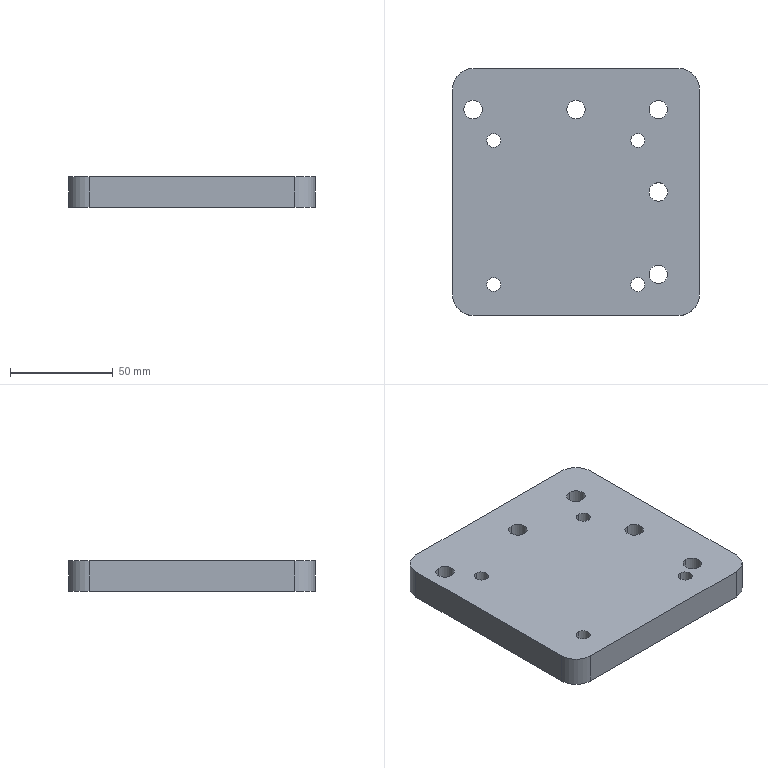Component | SolidWorks | CasterFixingPlate3-2 | 1 solid | 43 faces | box 120 x 120 x 15 mm | volume 202899 mm3 | cylinder 32 | plane 11 | commonest cylinder face diameters 15 x10 9 x10 6.8 x8 20 x4
build123d program:
from build123d import *

# Parameters (mm, degrees)
SKETCH1_W                                       = 240
SKETCH1_H                                       = 120
BOSS_EXTRUDE1_DEPTH                             = 15
M8_HEX_SOCKET_HEAD_CAP_SCREW_CBORE1_D           = 9
M8_HEX_SOCKET_HEAD_CAP_SCREW_CBORE1_DEPTH       = 20
M8_HEX_SOCKET_HEAD_CAP_SCREW_CBORE1_CBORE_D     = 15
M8_HEX_SOCKET_HEAD_CAP_SCREW_CBORE1_CBORE_DEPTH = 8.6
M8_HEX_SOCKET_HEAD_CAP_SCREW_CBORE1_TIP         = 2.704
FILLET1_R                                       = 10
M8_TAPPED_HOLE1_D                               = 6.8
M8_TAPPED_HOLE1_DEPTH                           = 22.25
M8_TAPPED_HOLE1_TIP                             = 2.043
M8_HEX_SOCKET_HEAD_CAP_SCREW_CBORE2_D           = 9
M8_HEX_SOCKET_HEAD_CAP_SCREW_CBORE2_DEPTH       = 27.5
M8_HEX_SOCKET_HEAD_CAP_SCREW_CBORE2_CBORE_D     = 15
M8_HEX_SOCKET_HEAD_CAP_SCREW_CBORE2_CBORE_DEPTH = 8.6
M8_HEX_SOCKET_HEAD_CAP_SCREW_CBORE2_TIP         = 2.704
SKETCH8_W                                       = 120
SKETCH8_H                                       = 120
CUT_EXTRUDE1_DEPTH                              = 73
FILLET2_R                                       = 10
M8_TAPPED_HOLE2_D                               = 6.8
M8_TAPPED_HOLE2_DEPTH                           = 22.25
M8_TAPPED_HOLE2_TIP                             = 2.043


with BuildPart() as part:
    # Sketch1 → Boss-Extrude1 (new body)
    with BuildSketch(Plane.XY):
        Rectangle(SKETCH1_W, SKETCH1_H)
    extrude(amount=BOSS_EXTRUDE1_DEPTH)

    # M8 Hex Socket Head Cap Screw CBORE1
    with Locations(Plane.XY.offset(15)):
        with Locations((-60, 40), (-20, 40), (20, 40), (60, 40), (-100, 40), (100, 40)):
            CounterBoreHole(M8_HEX_SOCKET_HEAD_CAP_SCREW_CBORE1_D / 2, M8_HEX_SOCKET_HEAD_CAP_SCREW_CBORE1_CBORE_D / 2, M8_HEX_SOCKET_HEAD_CAP_SCREW_CBORE1_CBORE_DEPTH, depth=M8_HEX_SOCKET_HEAD_CAP_SCREW_CBORE1_DEPTH)
            with Locations((0, 0, -(M8_HEX_SOCKET_HEAD_CAP_SCREW_CBORE1_DEPTH + M8_HEX_SOCKET_HEAD_CAP_SCREW_CBORE1_TIP / 2))):  # 118° drill point
                Cone(0, M8_HEX_SOCKET_HEAD_CAP_SCREW_CBORE1_D / 2, M8_HEX_SOCKET_HEAD_CAP_SCREW_CBORE1_TIP, mode=Mode.SUBTRACT)

    # Fillet1
    fillet1_edges = [part.edges().sort_by_distance(p)[0] for p in [
        (-120, 60, 7.5),
        (120, 60, 7.5),
        (120, -60, 7.5),
        (-120, -60, 7.5),
    ]]
    fillet(fillet1_edges, radius=FILLET1_R)

    # M8 Tapped Hole1
    with Locations(Plane.XY.offset(15)):
        with Locations((-35, 30), (-35, -40), (35, 30), (35, -40)):
            Hole(M8_TAPPED_HOLE1_D / 2, depth=M8_TAPPED_HOLE1_DEPTH)
            with Locations((0, 0, -(M8_TAPPED_HOLE1_DEPTH + M8_TAPPED_HOLE1_TIP / 2))):  # 118° drill point
                Cone(0, M8_TAPPED_HOLE1_D / 2, M8_TAPPED_HOLE1_TIP, mode=Mode.SUBTRACT)

    # M8 Hex Socket Head Cap Screw CBORE2
    with Locations(Plane.XY.offset(15)):
        with Locations((-20, 0), (-20, -50), (20, 0), (20, -50)):
            CounterBoreHole(M8_HEX_SOCKET_HEAD_CAP_SCREW_CBORE2_D / 2, M8_HEX_SOCKET_HEAD_CAP_SCREW_CBORE2_CBORE_D / 2, M8_HEX_SOCKET_HEAD_CAP_SCREW_CBORE2_CBORE_DEPTH, depth=M8_HEX_SOCKET_HEAD_CAP_SCREW_CBORE2_DEPTH)
            with Locations((0, 0, -(M8_HEX_SOCKET_HEAD_CAP_SCREW_CBORE2_DEPTH + M8_HEX_SOCKET_HEAD_CAP_SCREW_CBORE2_TIP / 2))):  # 118° drill point
                Cone(0, M8_HEX_SOCKET_HEAD_CAP_SCREW_CBORE2_D / 2, M8_HEX_SOCKET_HEAD_CAP_SCREW_CBORE2_TIP, mode=Mode.SUBTRACT)

    # Sketch8 → Cut-Extrude1 (cut)
    with BuildSketch(Plane.XY.offset(15)):
        with Locations((60, 0)):
            Rectangle(SKETCH8_W, SKETCH8_H)
    extrude(amount=-CUT_EXTRUDE1_DEPTH, mode=Mode.SUBTRACT)

    # Fillet2
    fillet2_edges = [part.edges().sort_by_distance(p)[0] for p in [
        (0, -60, 7.5),
        (0, 60, 7.5),
    ]]
    fillet(fillet2_edges, radius=FILLET2_R)

    # M8 Tapped Hole2
    with Locations(Plane.XY.offset(15)):
        with Locations((-105, 30), (-105, -40)):
            Hole(M8_TAPPED_HOLE2_D / 2, depth=M8_TAPPED_HOLE2_DEPTH)
            with Locations((0, 0, -(M8_TAPPED_HOLE2_DEPTH + M8_TAPPED_HOLE2_TIP / 2))):  # 118° drill point
                Cone(0, M8_TAPPED_HOLE2_D / 2, M8_TAPPED_HOLE2_TIP, mode=Mode.SUBTRACT)


solid = part.part

# Placed as in the assembly
solid = solid.moved(Location((-1228.352, -468.217, -96.285), (180, 0, -90)))